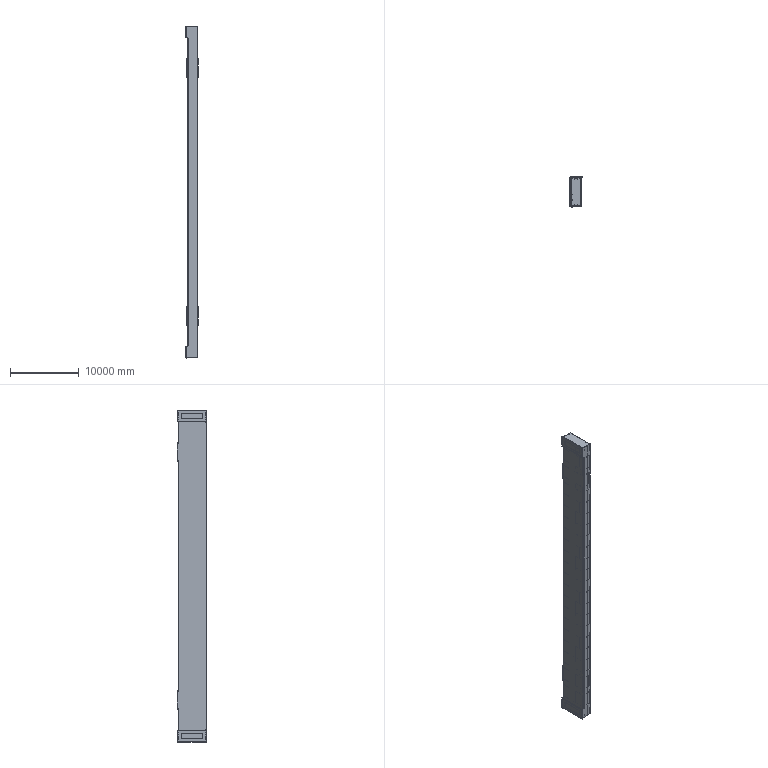Component | SolidWorks | MainBeam-1 | 1 solid | 1906 faces | volume 38220713452 mm3 | plane 1375 | cylinder 404 | spline 127 | commonest cylinder face diameters 40 x288 200 x108 100 x8